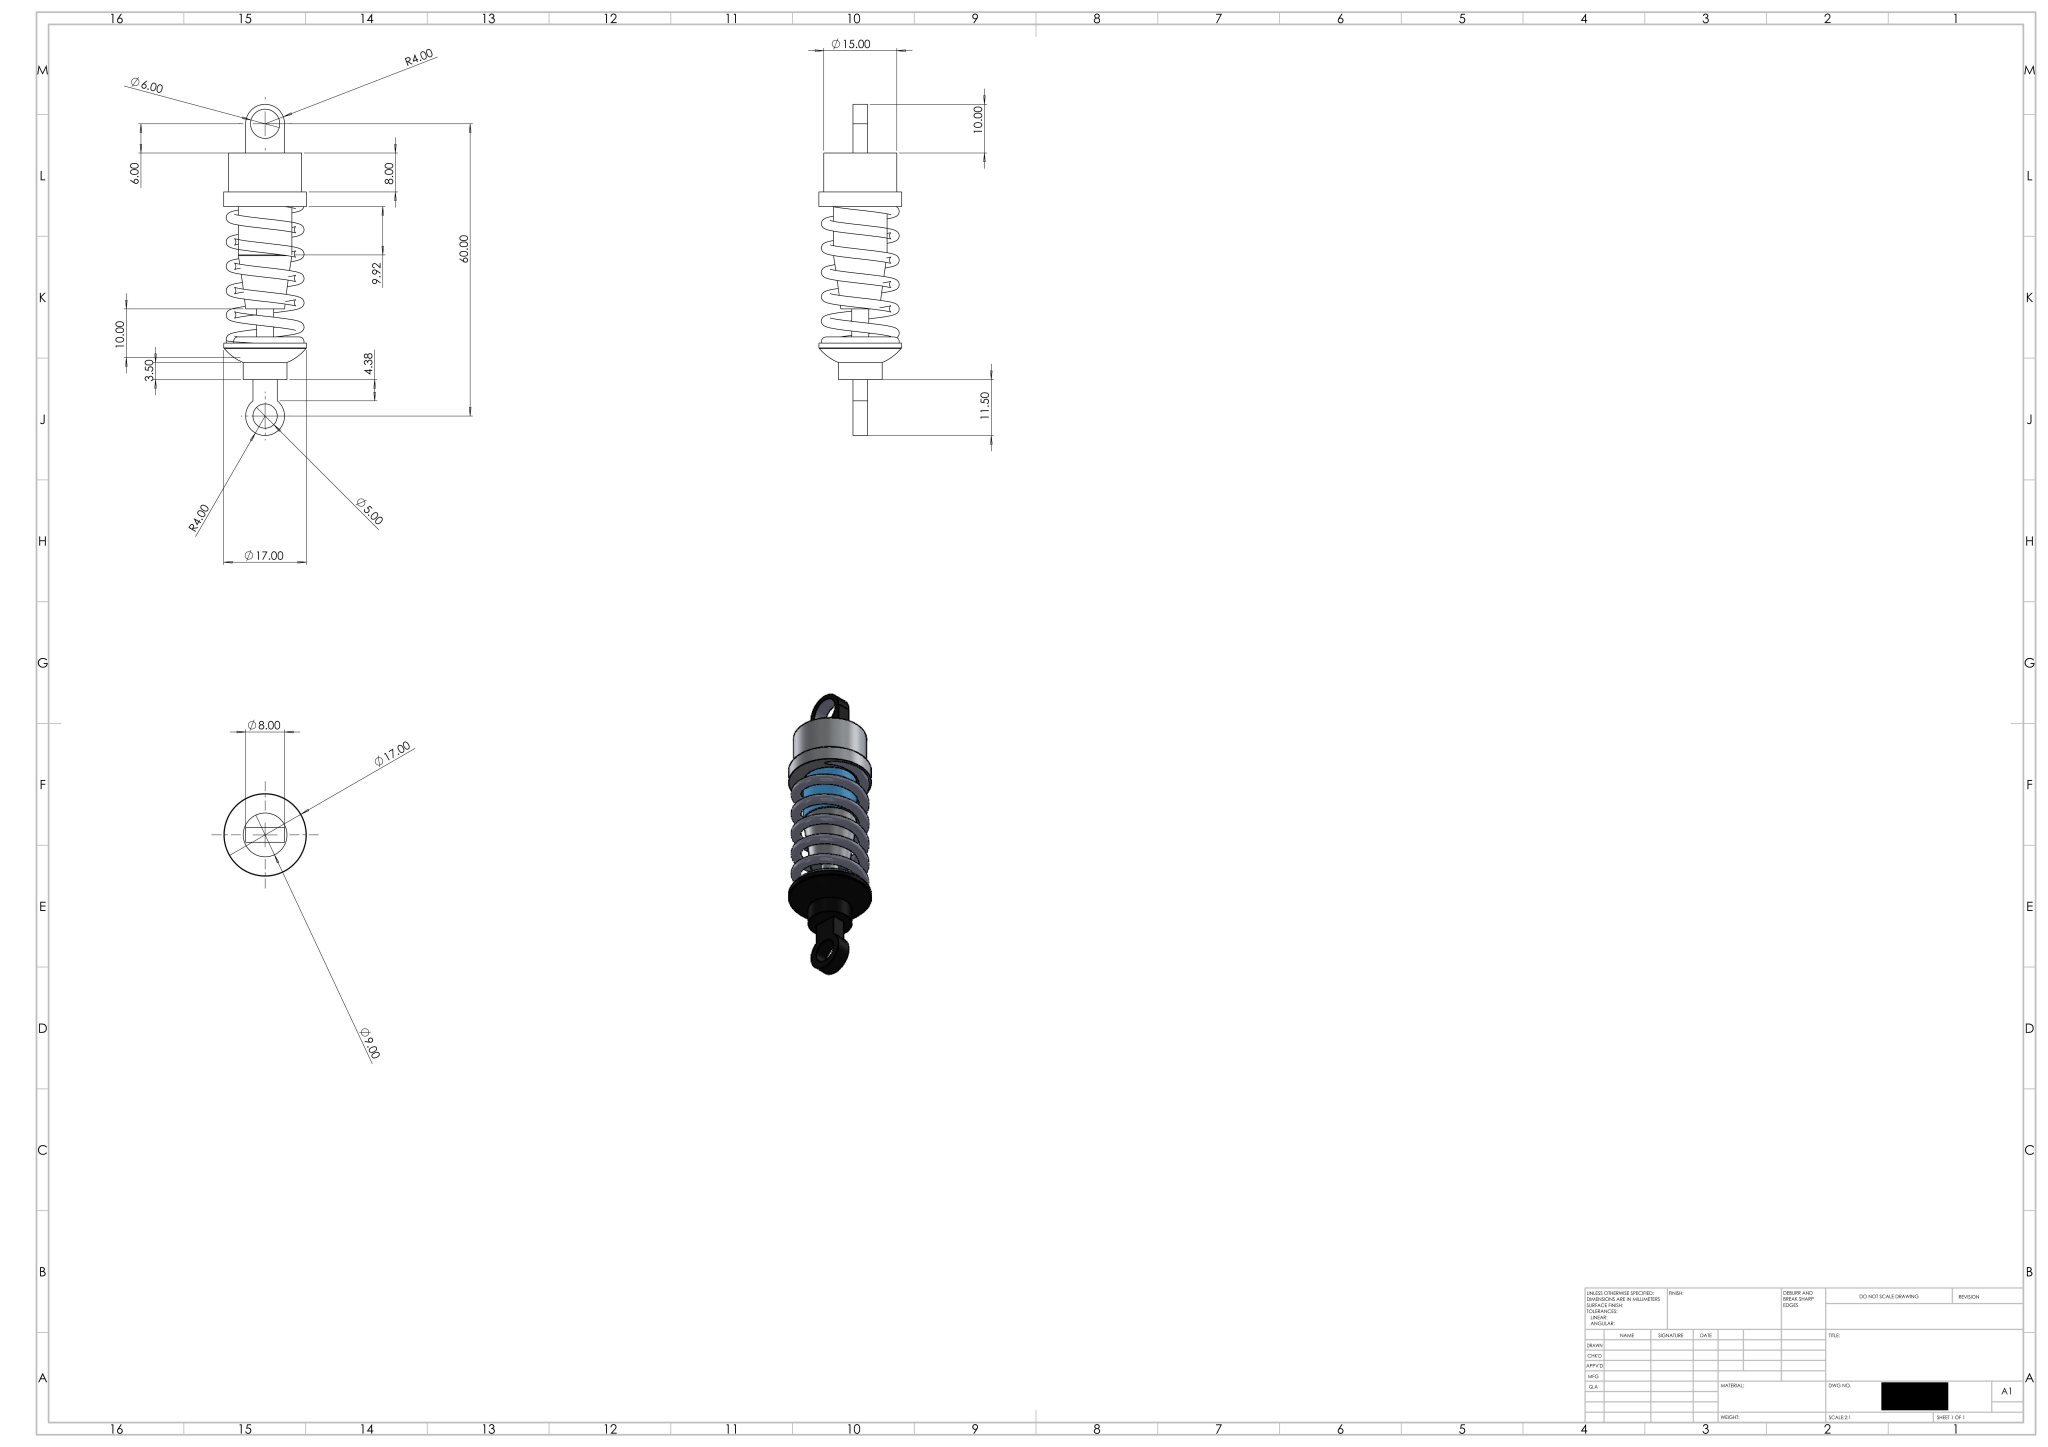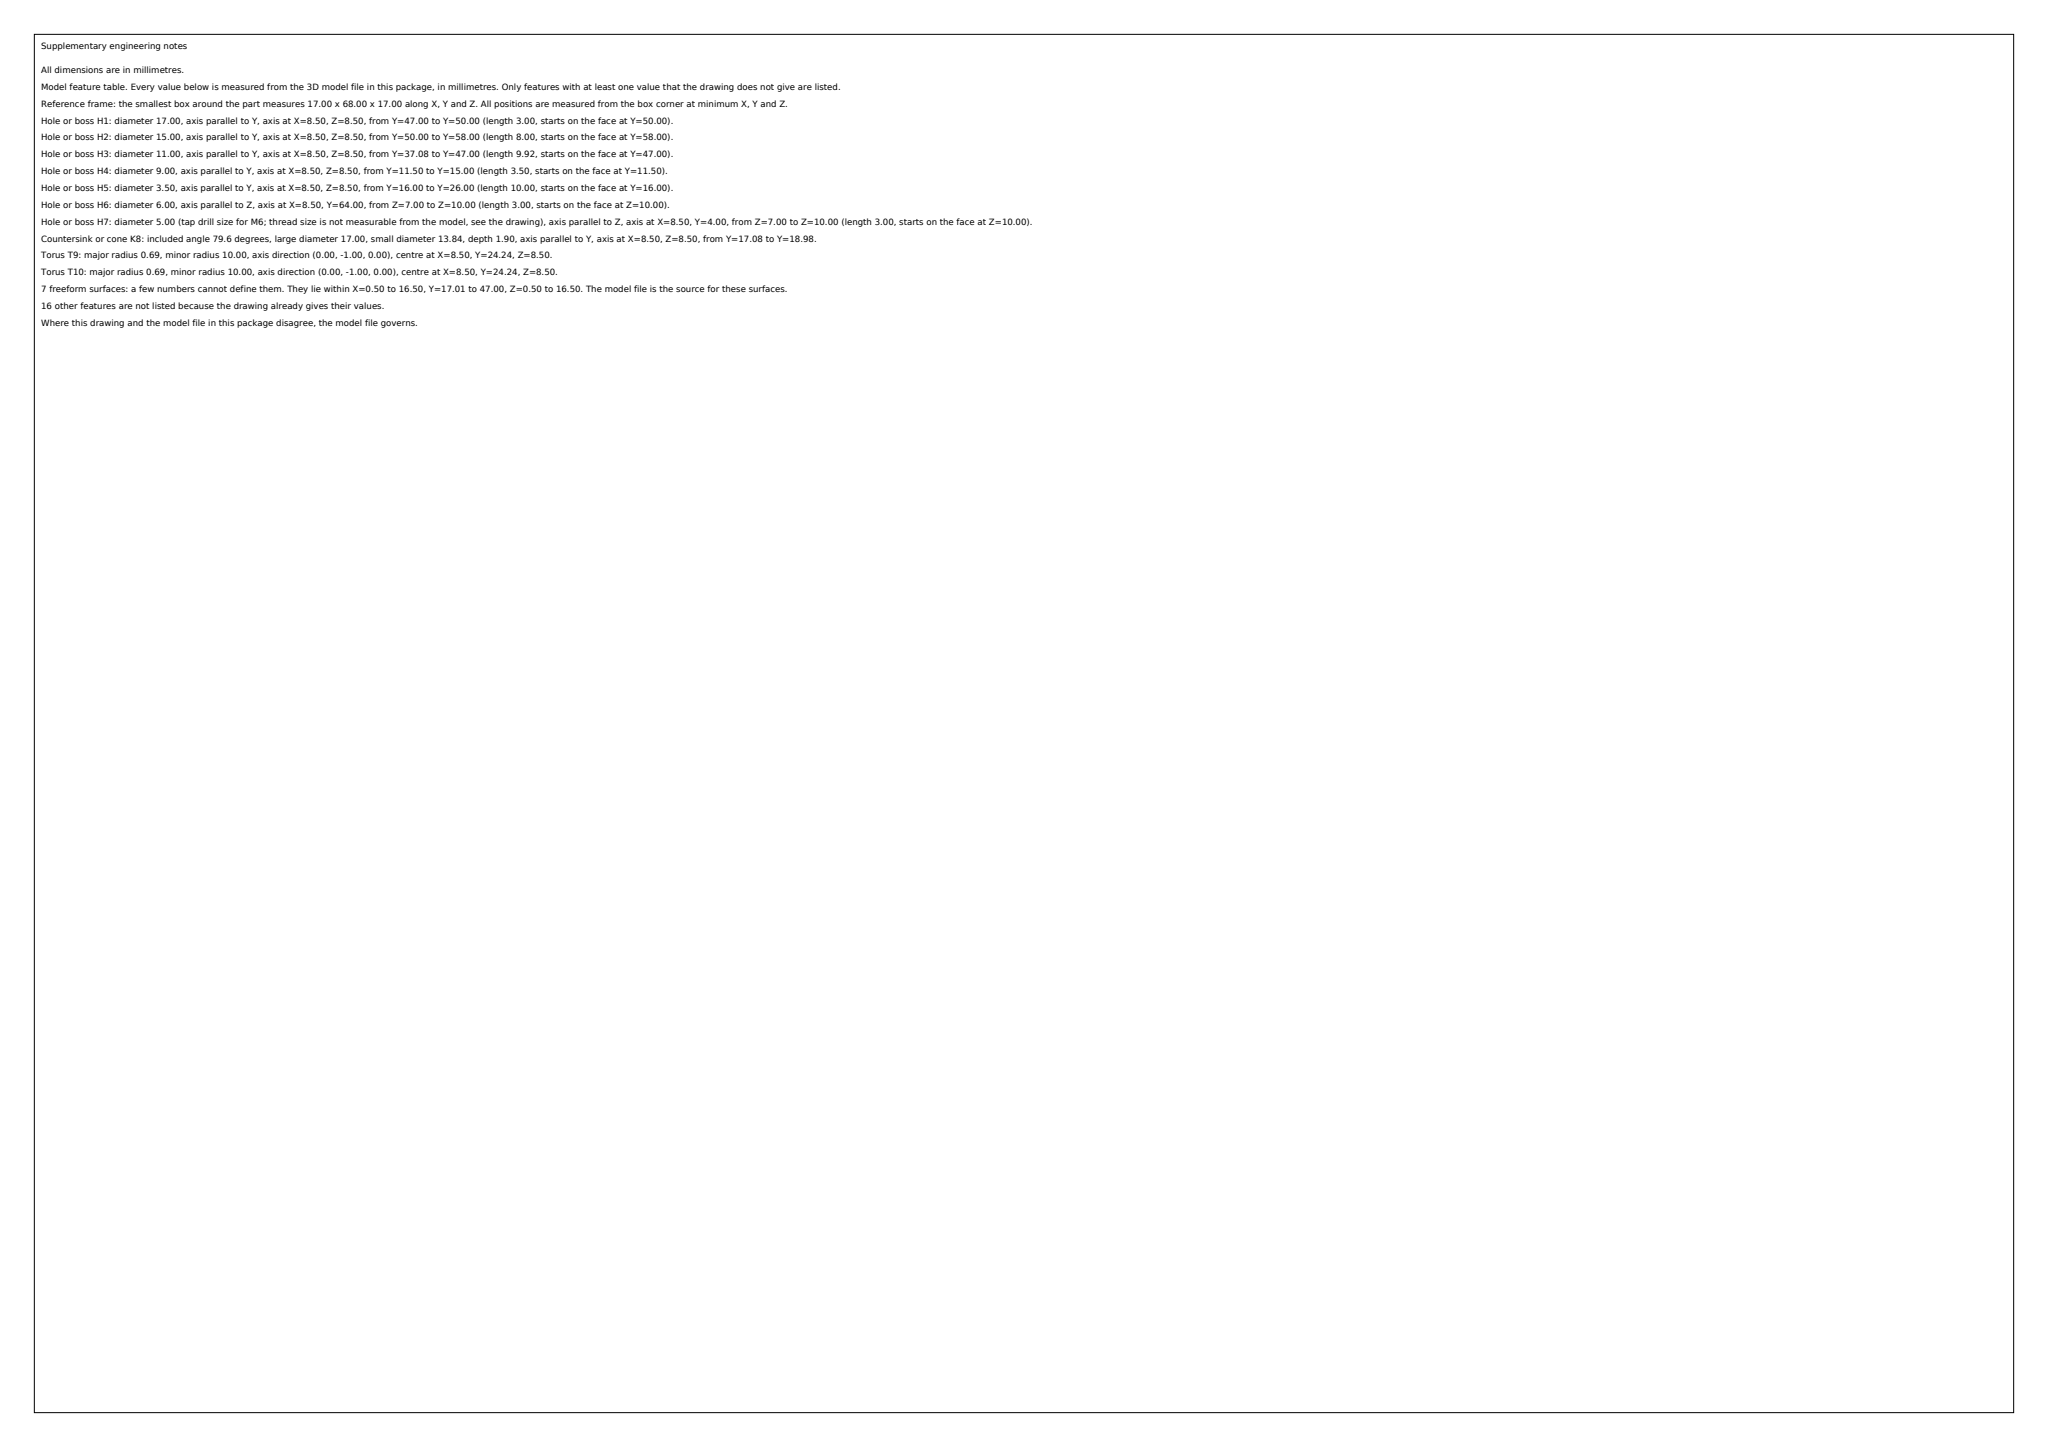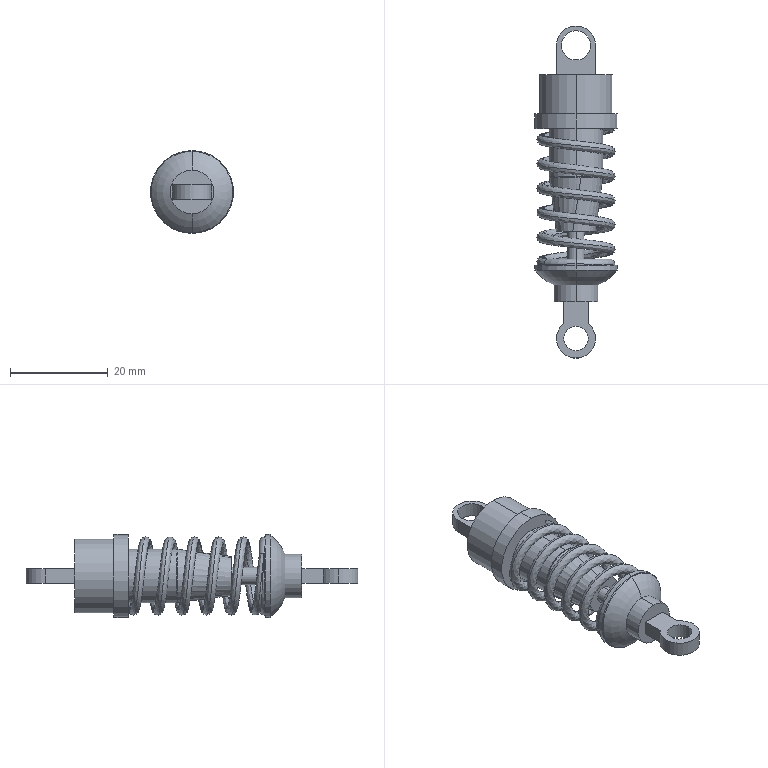Part | SolidWorks | mm | 1 solid | 61 faces | box 17 x 68 x 17 mm | volume 5511 mm3 | cylinder 18 | plane 15 | torus 14 | cone 7 | spline 7 | commonest cylinder face diameters 8 x4 5 x2 9 x2 3.5 x2 11 x2 6 x2 17 x2 15 x2